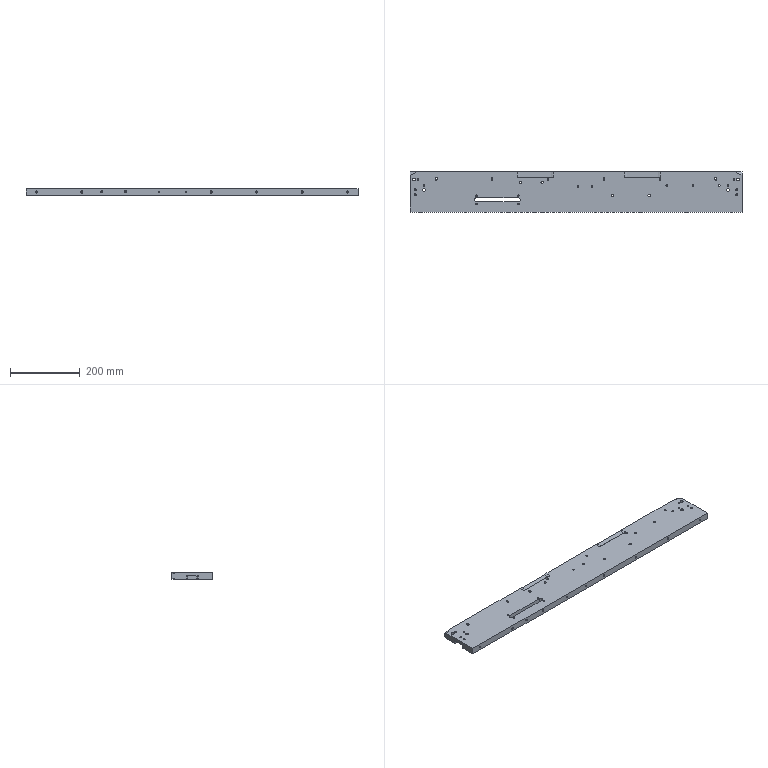Component | SolidWorks | --MA18S20041SidePlate1-1 | 1 solid | 209 faces | volume 2007453 mm3 | cylinder 123 | plane 66 | cone 20 | commonest cylinder face diameters 5 x52 4.2 x20 6 x16 10 x12 8 x8 6.8 x8 50 x4 11 x3